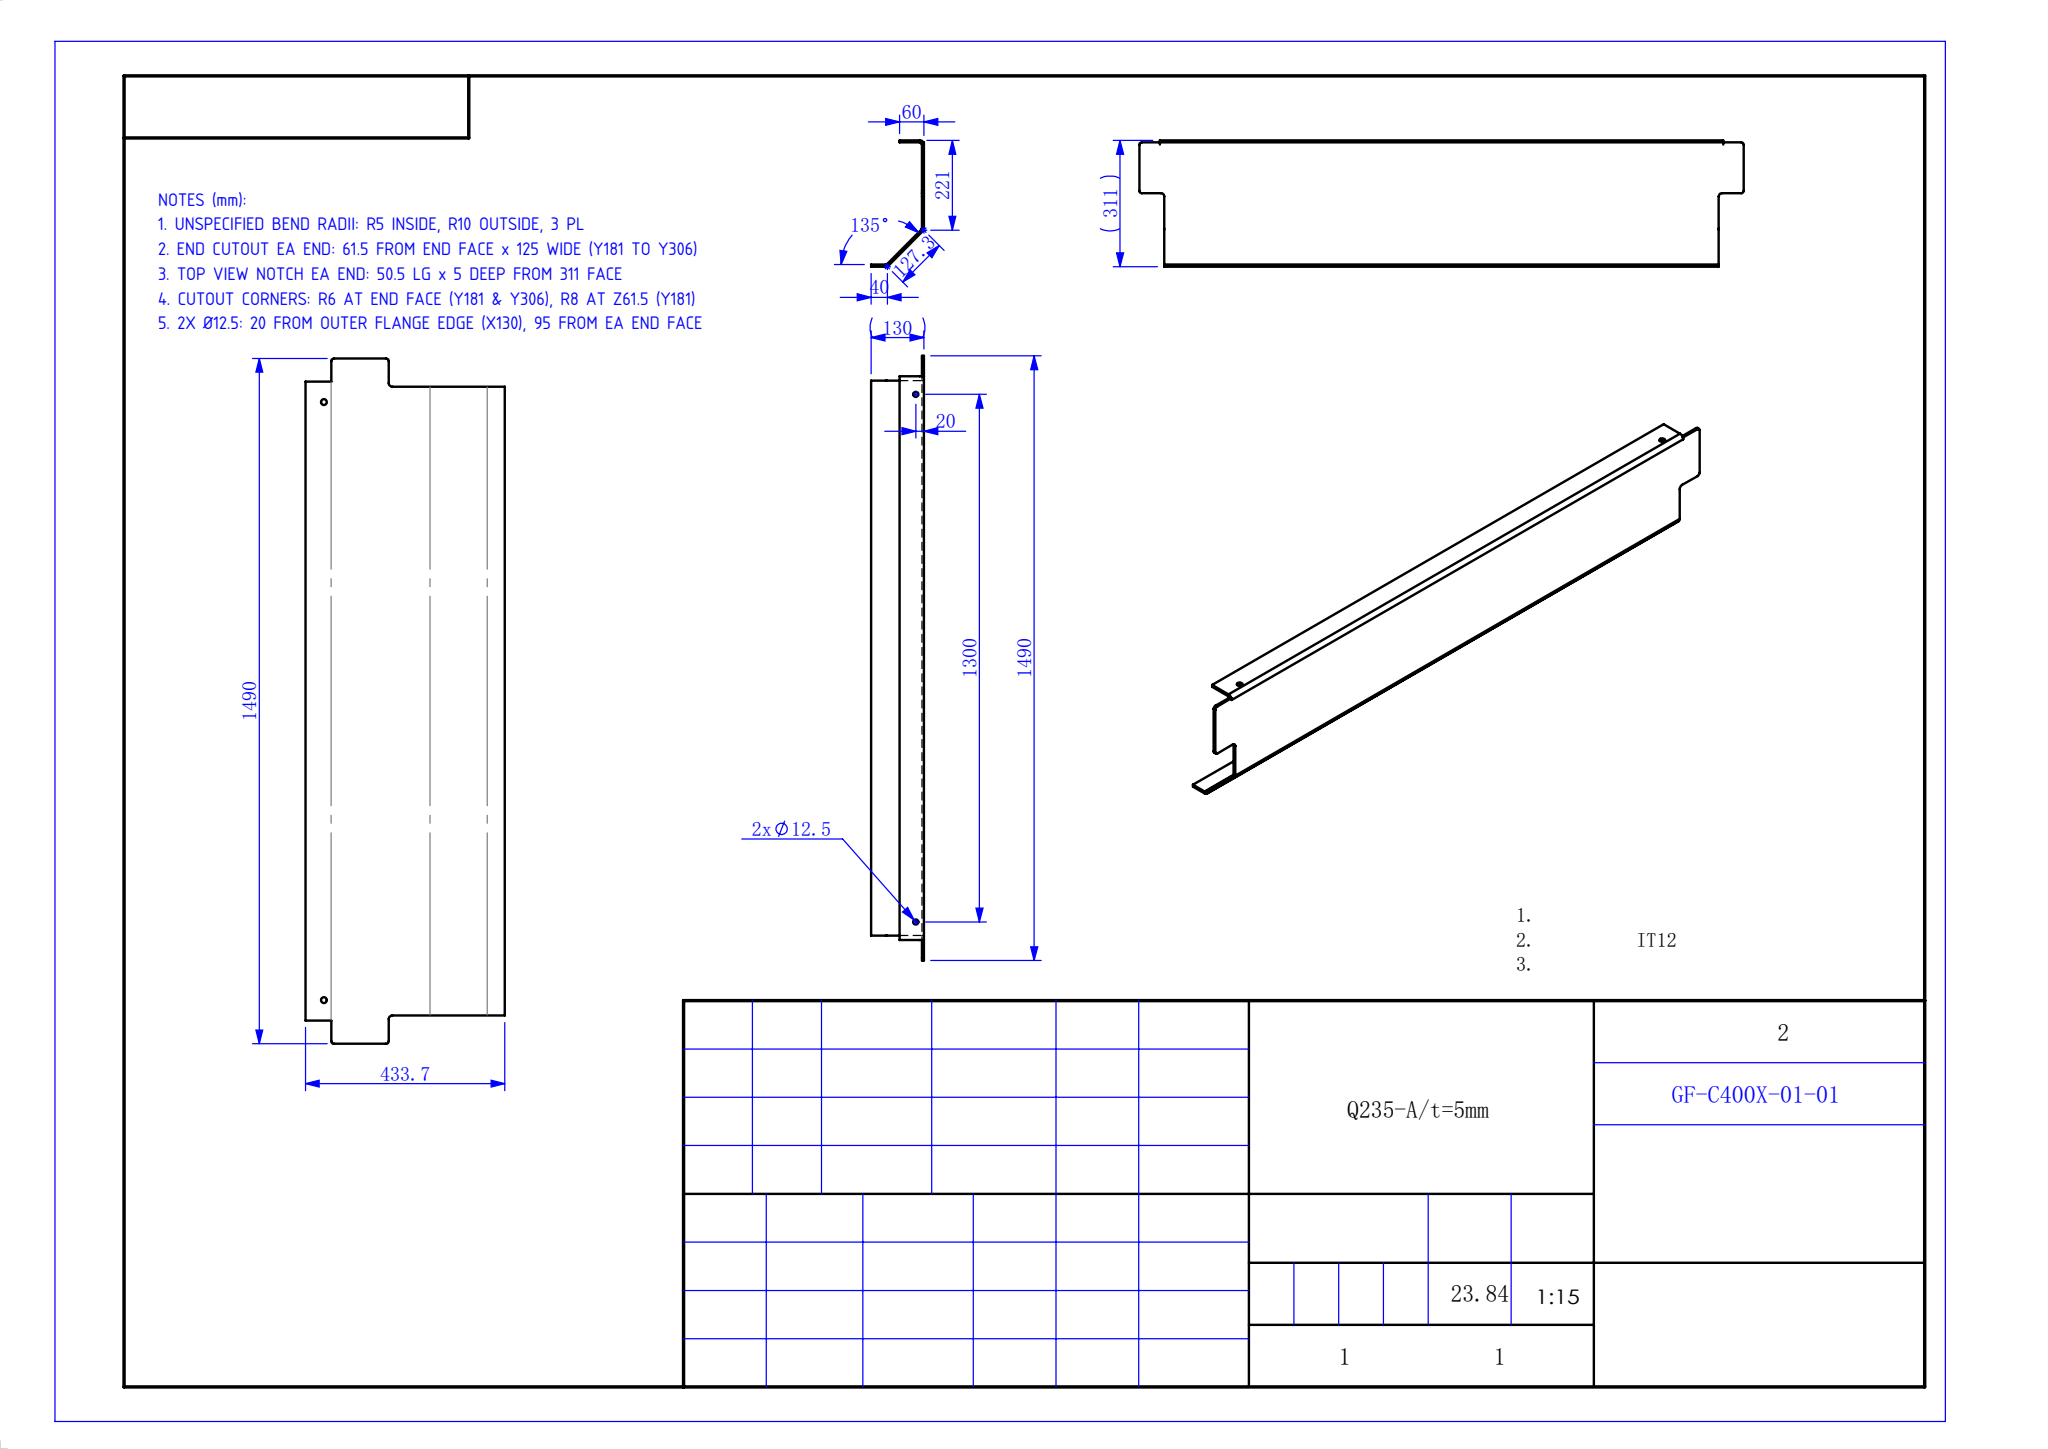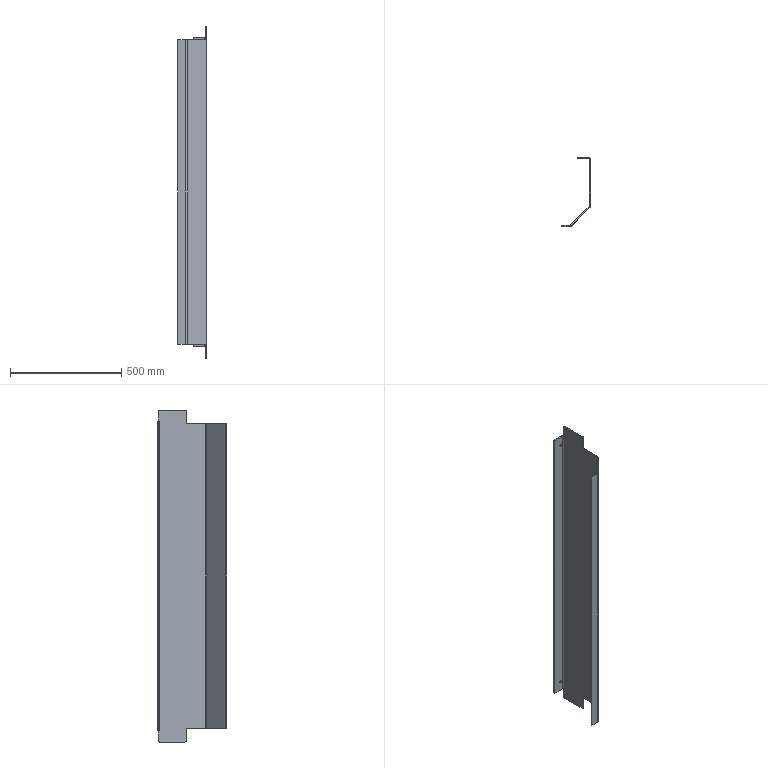Part | SolidWorks | mm | 1 solid | 40 faces | box 130 x 311 x 1490 mm | volume 3056965 mm3 | plane 24 | cylinder 16 | commonest cylinder face diameters 12.5 x4 12 x4 20 x3 10 x3 16 x2
Drawing notes:
UNSPECIFIED BEND RADII: R5 INSIDE, R10 OUTSIDE, 3 PL | from the solid: Z-axis cyls dia 10 & dia 20 at (35.86,10), (120,94.14), (120,301) = 3 bends, IR5/OR10
END CUTOUT EA END: 61.5 FROM END FACE x 125 WIDE (Y181 TO Y306) | from the solid: z planes 61.5 & 1428.5 with y planes 181 & 306; bbox z=1490
TOP VIEW NOTCH EA END: 50.5 LG x 5 DEEP FROM 311 FACE | from the solid: z planes 50.5 & 1439.5 (x3) with y planes 306 & 311, bbox y=311
CUTOUT CORNERS: R6 AT END FACE (Y181 & Y306), R8 AT Z61.5 (Y181) | from the solid: dia 12 x-cyls at y187/z6, y300/z6, y187/z1484, y300/z1484; dia 16 x-cyls at y173/z53.5 & z1436.5
2X Ø12.5: 20 FROM OUTER FLANGE EDGE (X130), 95 FROM EA END FACE | from the solid: dia 12.5 y-axis holes at x=110 (130-110=20), z=95 & 1395 (1490-1395=95), 1300 apart